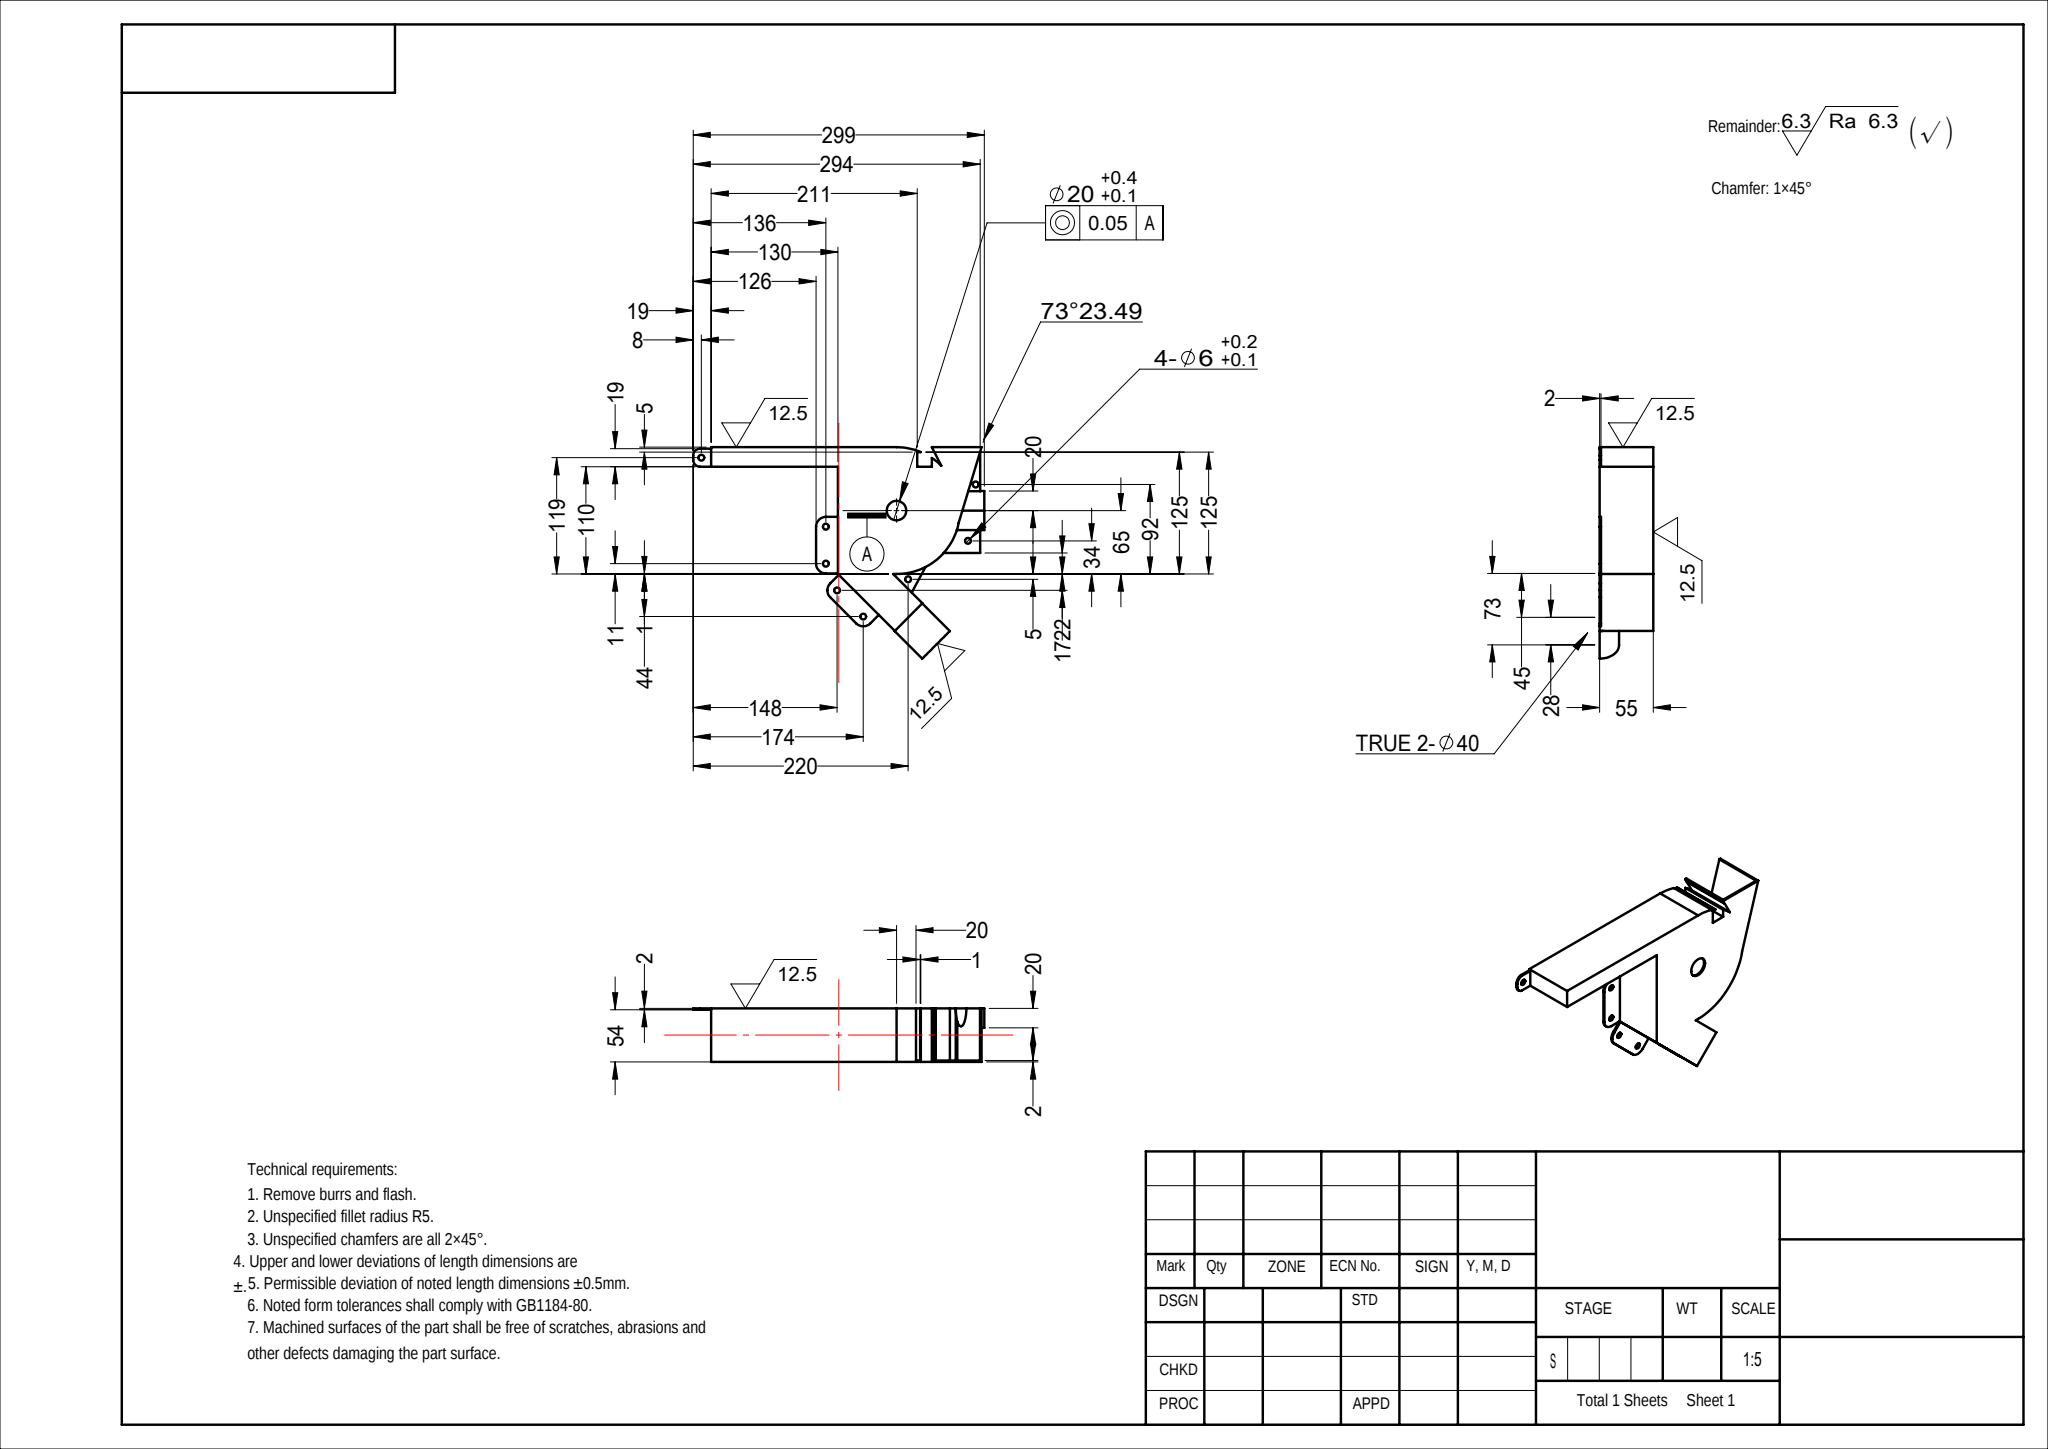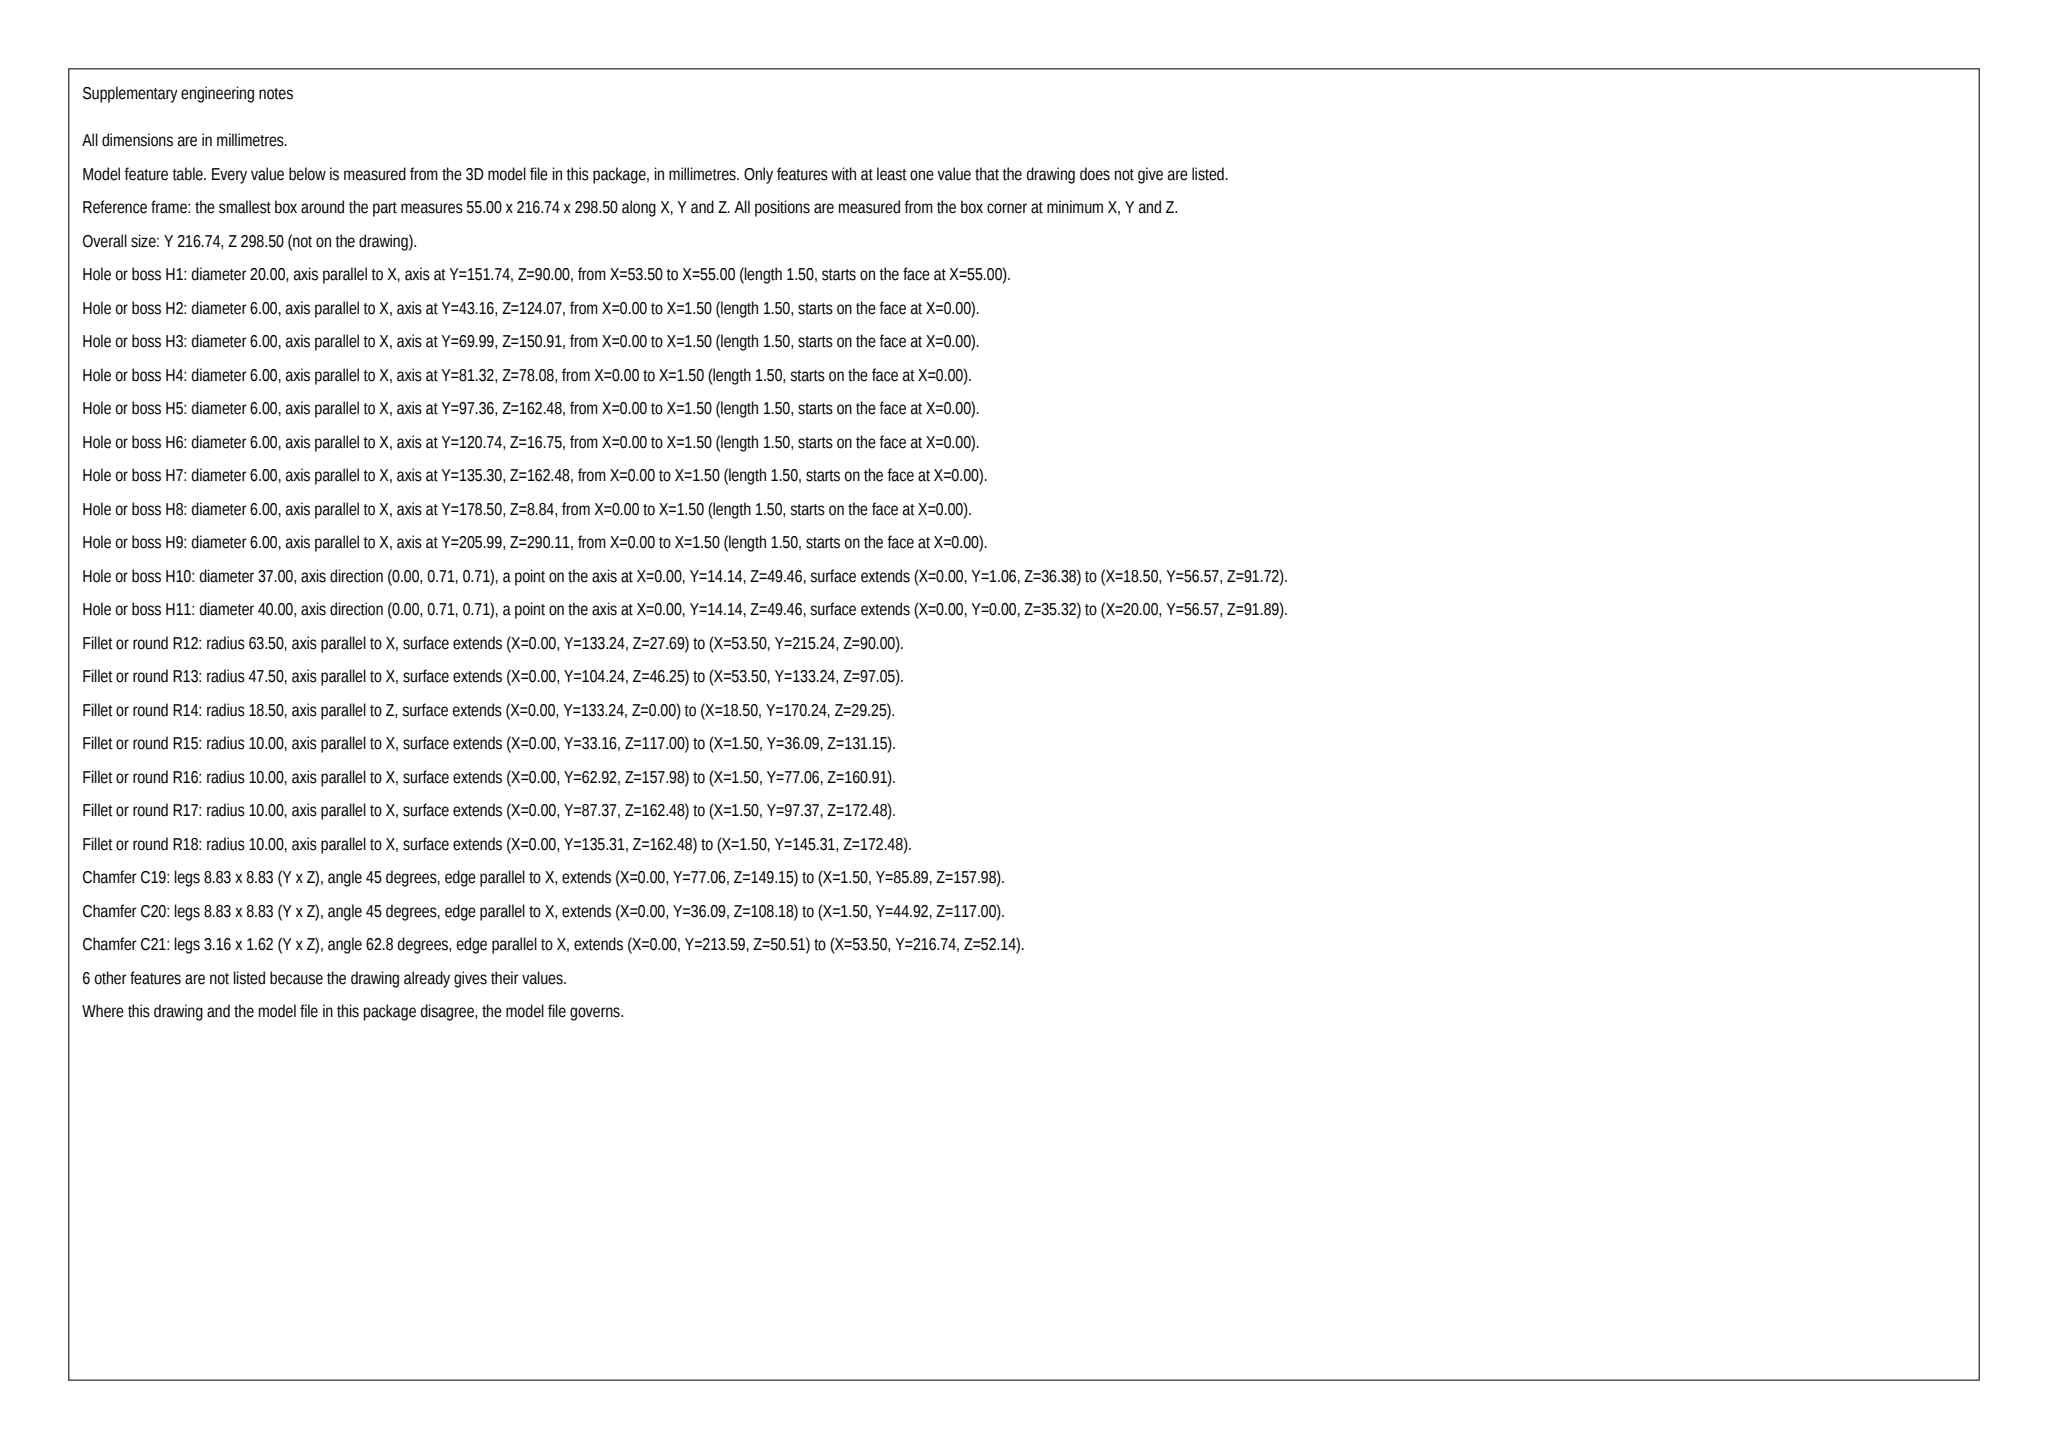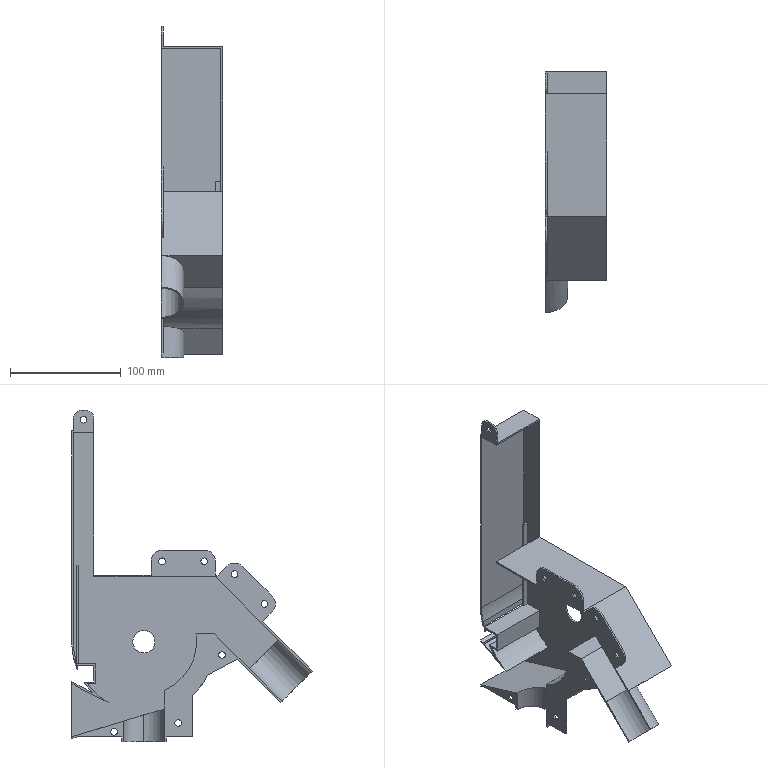Part | SolidWorks | mm | 1 solid | 105 faces | box 55 x 216.74 x 298.5 mm | volume 166772 mm3 | plane 67 | cylinder 38 | commonest cylinder face diameters 6 x16 20 x7 37 x3 127 x3 40 x3 130 x3 14 x2 95 x1